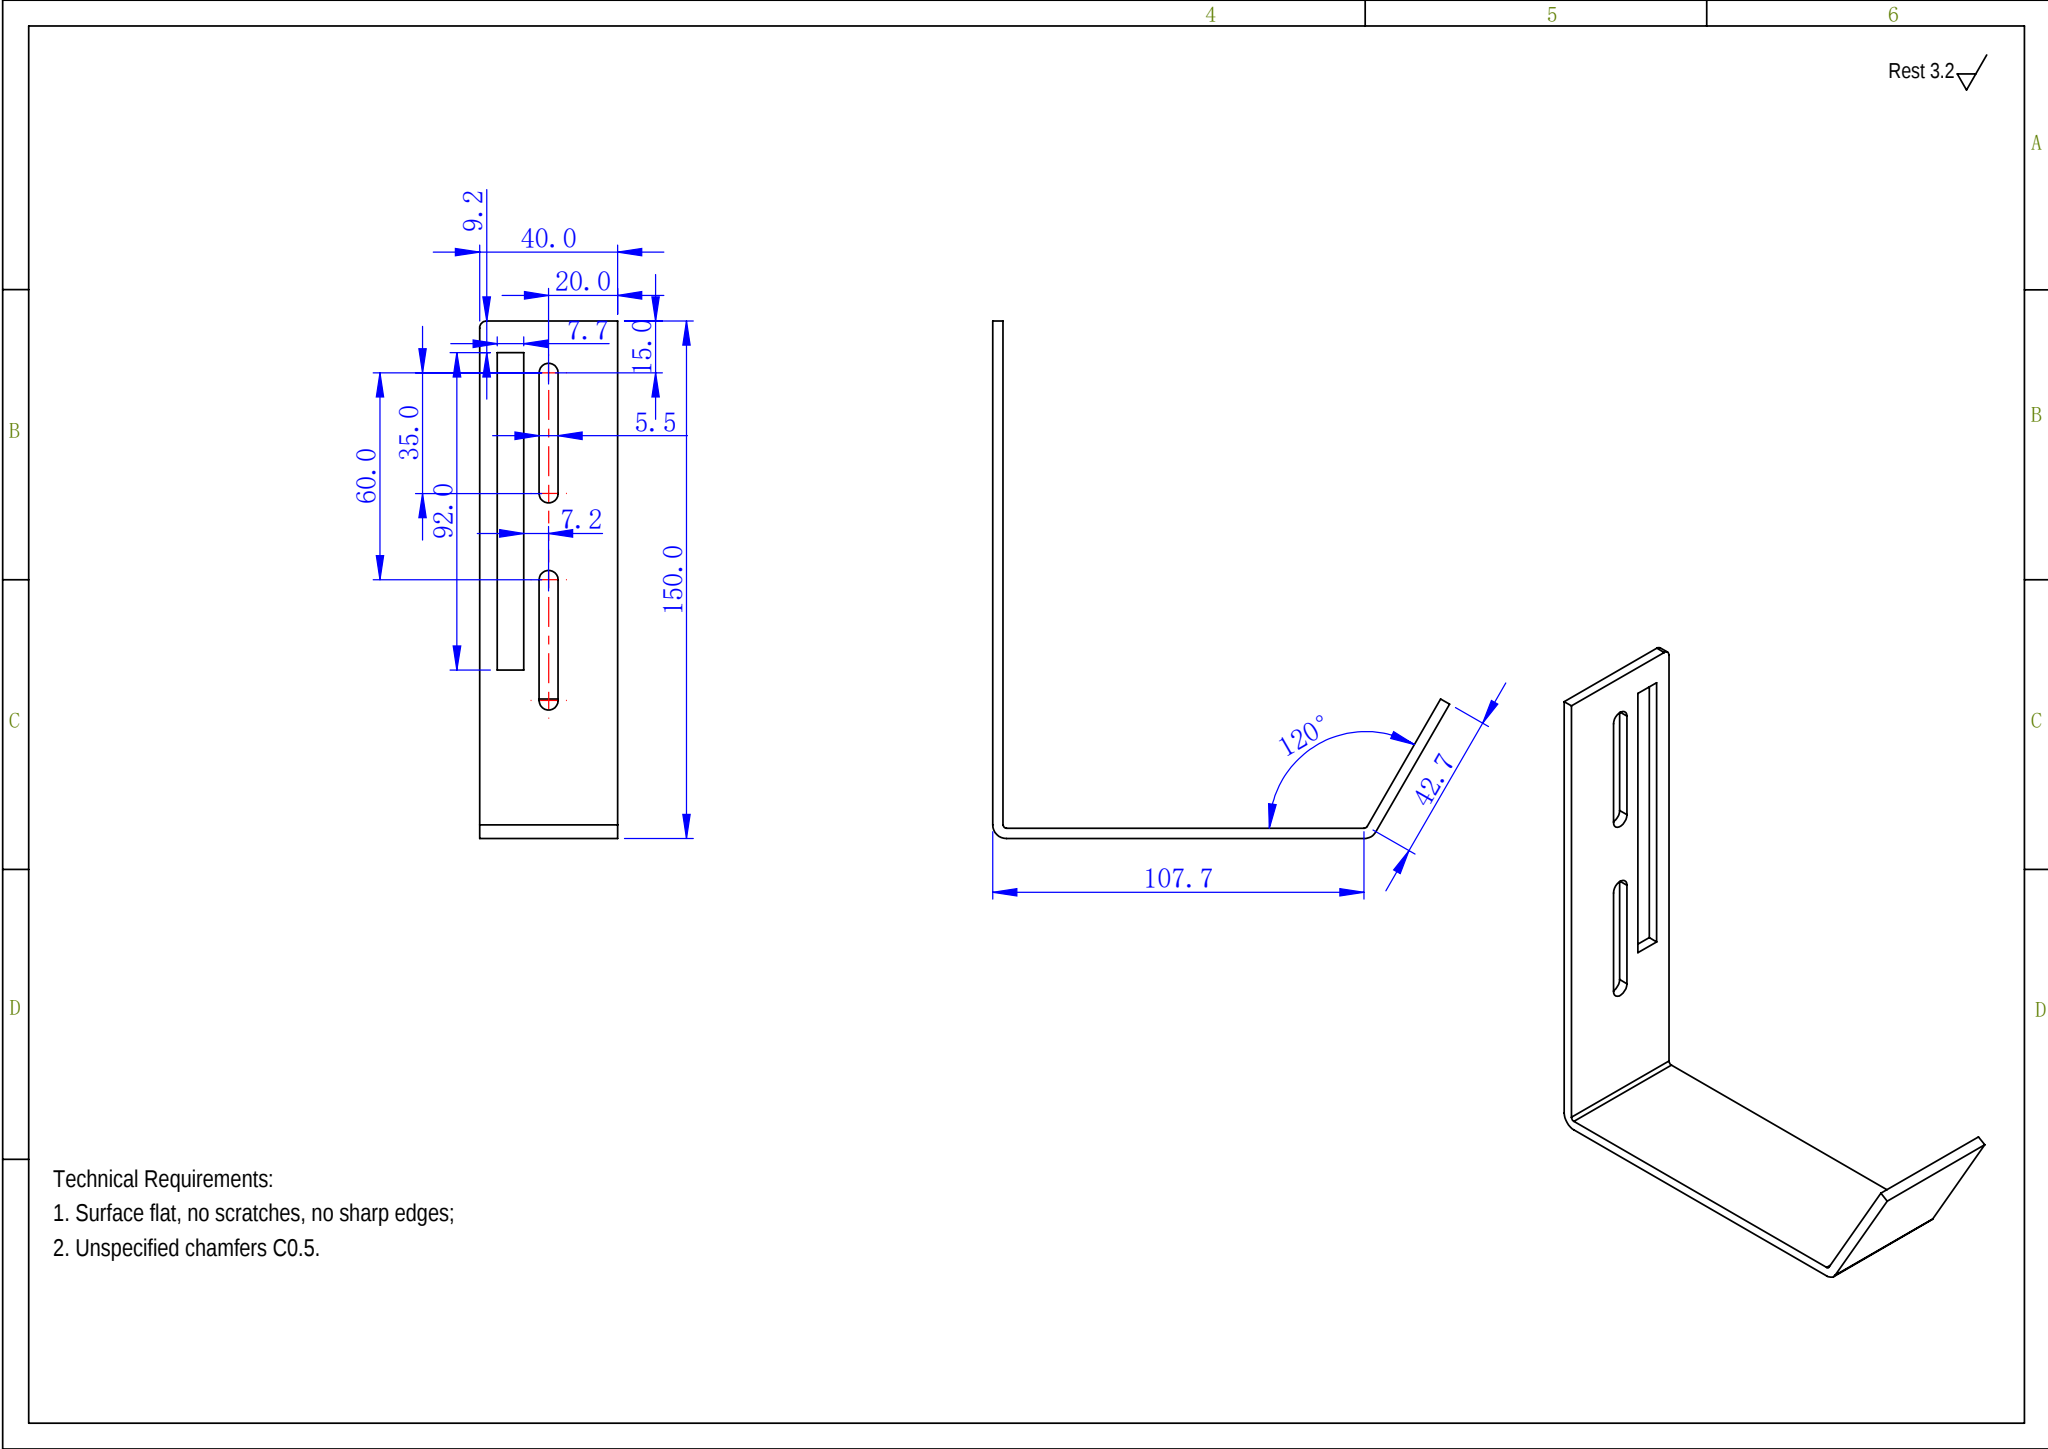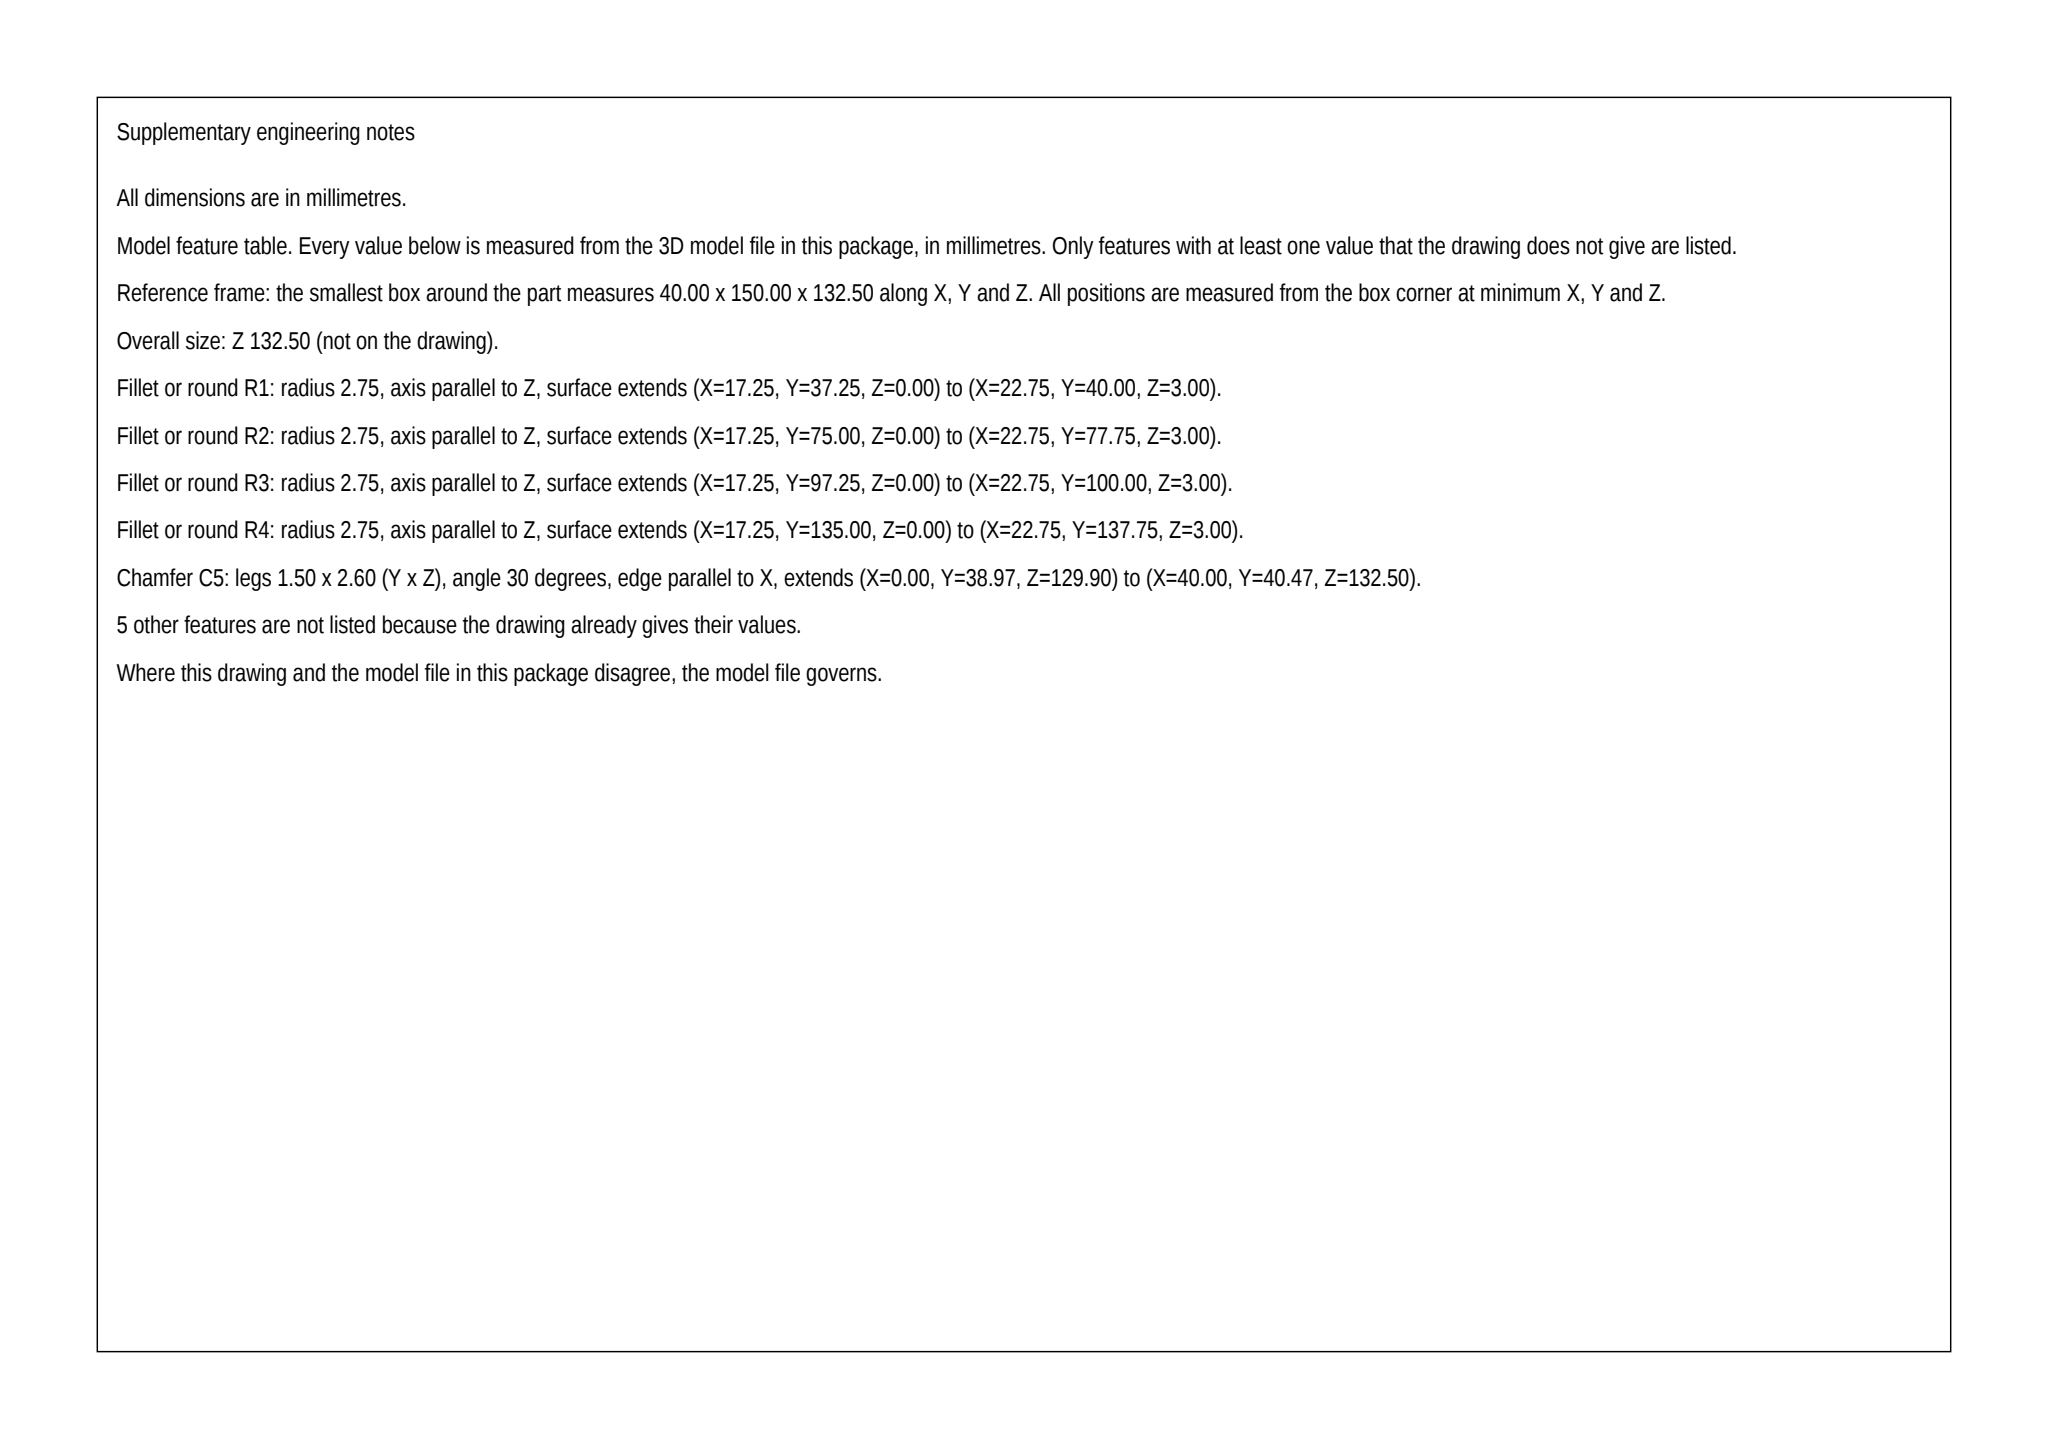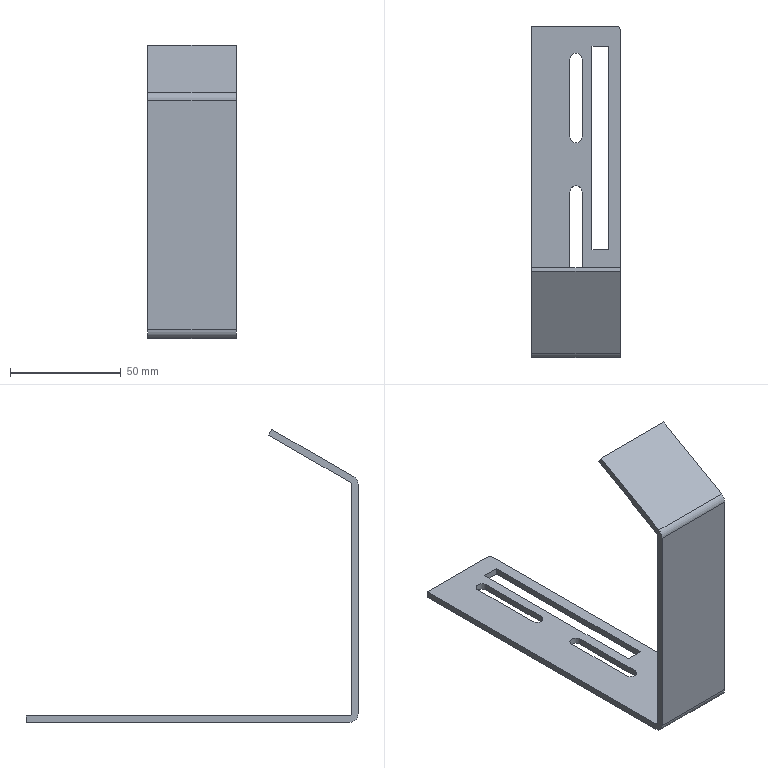Part | SolidWorks | mm | 1 solid | 27 faces | box 40 x 150 x 132.5 mm | volume 32451 mm3 | plane 18 | cylinder 9 | commonest cylinder face diameters 5.5 x4 2 x2 8 x2 4 x1